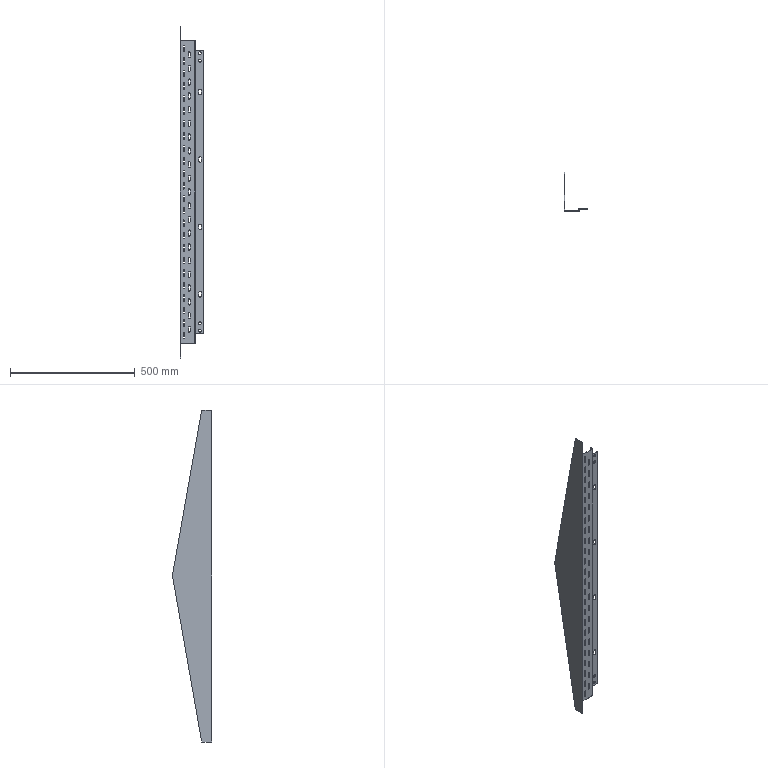Component | SolidWorks | Assembly2-1_TopPlateSideSealingPlate-2 | 1 solid | 245 faces | volume 367407 mm3 | plane 129 | cylinder 116 | commonest cylinder face diameters 6 x90 11 x20 3.4 x3 0.4 x3